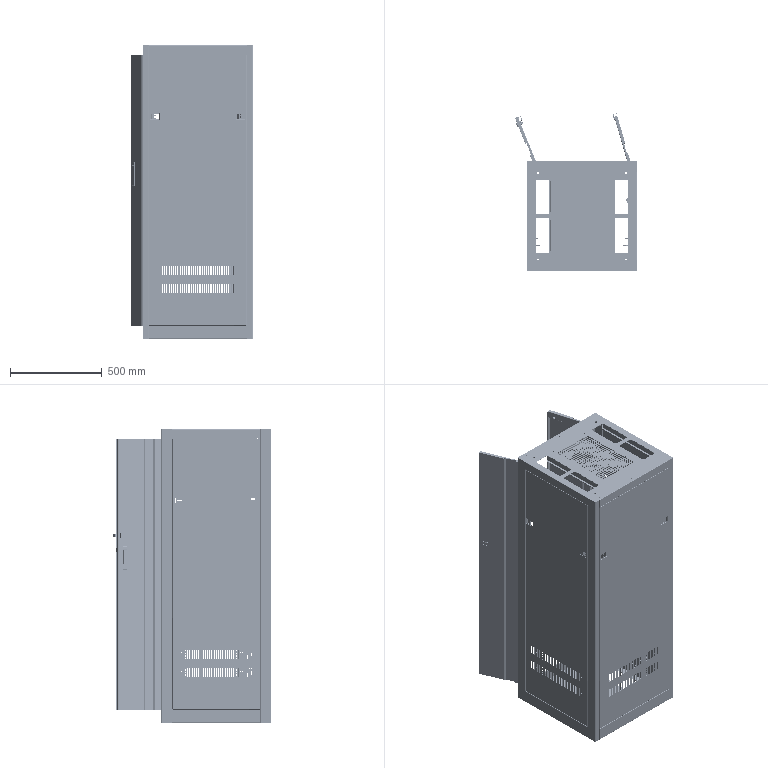Assembly | SolidWorks | mm | 61 component files | 61 solids | 10050 faces | box 662.77 x 864.74 x 1600 mm | volume 9328341 mm3 | plane 8344 | cylinder 1611 | spline 57 | sphere 16 | torus 14 | cone 8 | commonest cylinder face diameters 6 x533 2 x236 6.5 x162 1 x128 5 x74 9.2 x64 6.1 x52 4.5 x28
Bill of materials:
Base | 1 |  | Square, tray-like sheet-metal base plate. Formed channel walls run along two opposite edges and stop short of the corners, leaving gaps. The base has two long rounded-rectangle cutouts, round holes near the corners and small pierced holes.
Bracket1 | 4 |  | Long, straight Z-section profile of uniform cross-section: two parallel flanges joined by a web, with rounded bends.
Column | 4 |  | Long, slender formed sheet-metal profile with a multi-bend, stepped hat- or omega-like open cross-section. It has a row of small holes along its length and small notched tabs at one end.
FanMountingPlate | 1 |  | Rectangular, shallow open tray or box with vertical side walls and outward perimeter flanges. The base has two large circular cutouts, a small square cutout between them, and round holes.
2 | 1 |  | Long, narrow sheet-metal strip formed into a shallow channel (C/U) profile. The web has a repeating pattern of small square holes with adjacent slots along the full length.
CopperBarFixingClamp | 2 |  | Compact rectangular block with one rounded end. A deep slot along its length splits it into two parallel jaws (clevis- or fork-like), and a round through-hole passes across both jaws near the rounded end.
GroundingCopperBar | 1 |  | Very thin, flat rectangular plate or sheet panel, elongated in one direction, with tiny features along the long edges.
SC16-6 | 1 |  | Barrel-and-tongue lug-like part: a hollow cylindrical barrel joined through an offset transition to a flat rectangular tongue with rounded corners and one round through-hole.
GuidePlate | 4 |  | Long, straight formed rail with a stepped, hat-like cross-section and offset flanges. A row of square holes runs along the central raised section, and round holes sit near each end of both flanges.
Bolt | 2 |  | Solid round rod bent into a U or hairpin shape with two parallel legs of unequal length. The shorter leg has a circumferential groove or step near its end.
Bracket | 2 |  | Formed sheet-metal U or C bracket: a rectangular web with two parallel flanges bent at rounded corners. One flange has a round hole; each flange has a stepped notch giving a narrower tab at its free end.
EndCap1 | 2 |  | Long, formed sheet-metal channel with a multi-bend open profile (C-section with an extra offset return lip). The flanges have notched or stepped edges, there is a rectangular slot in the web near one end, and a small semicircular notch or hole sits at one end.
EndCap2 | 2 |  | Long, narrow formed sheet-metal channel or rail. It has an open, roughly C/Z-shaped cross-section with flanges that are offset from each other, stepped notches along the flange edges, and a small rectangular slot in the web near one end.
LeftDoor | 1 |  | Long thin-walled profile with a constant cross-section. The end view shows a multi-bend zigzag of mostly straight segments with short hooked returns at both ends. A small protruding rib or tab runs along one segment near one end.
LockWeldBracket | 1 |  | Hat-shaped (omega-profile) bent strip bracket. A central flat web has three round holes in a triangular pattern. Two side walls stand perpendicular to the web, and two outward-turned end flanges are coplanar with each other.
PadlockBracket | 1 |  | L-shaped bent plate bracket with two legs at roughly 90 degrees and a rounded bend. The shorter leg has three small round holes in a triangular pattern. The longer leg ends in a fully rounded end with one larger round hole.
Pin | 8 |  | Solid revolved pin or plug-like part. From one end it has a short cylindrical head, then a wider thin circular collar, then a cylindrical shank ending in a hemispherical (domed) tip.
Spring | 2 |  | Helical coil spring made of round wire. It has about 11 coils of uniform diameter, an open pitch, and plain cut ends that are not closed.
RearDoor | 1 |  | Thin flat rectangular panel. It has two small rectangular cutouts near the side edges toward one end, and two parallel rows of narrow elongated slots (vent-like) near the other end. Small round holes are visible on one narrow edge face.
ReinforcementPlate1 | 1 |  | Flat plate bracket whose outline has one chamfered (diagonally cut) corner. Two rectangular tabs on adjacent edges are bent up at about 90 degrees. The plate has two large round holes, several smaller round holes, and narrow rectangular slots cut in from the edges.
ReinforcementPlate2 | 1 |  | Flat plate bracket with one chamfered corner. Two rectangular tabs on adjacent edges are bent up at about 90 degrees. The plate has two large round holes, several smaller round holes, and narrow edge slots. The layout appears mirrored relative to unnamed part.
Latch | 1 |  | Bent flat strip with an S/Z-shaped jog made by two rounded bends, so the end segments are offset and run in parallel directions. One end segment has a square through-hole oriented as a diamond.
LockBody | 1 |  | Compact, blocky multi-feature part. A thin base plate or flange strip carries two raised rectangular blocks separated by a gap. One block has a chamfered or angled top. Shallow rectangular recesses are on the top face, and small round holes or bosses are on the side faces.
LowerRod | 1 |  | Long narrow flat strip with two jogged offsets along its length, so the middle and end sections step sideways. A small tab or barb-like protrusion sits at one end. The view along the length shows a T-shaped head over a narrower neck and a wider body.
UpperRod | 1 |  | Long, narrow flat strip with a joggle (offset bend) near one end. A short headed pin or stud sticks out from the face near the offset end.
LowerLinkRod1 | 1 |  | Very slender flat strip with a joggle near one end. One end has a small square hole and the other end is rounded with a small round hole.
Roller | 4 |  | Flat circular disc with one concentric through-hole, shaped like a washer or spacer. The outer edge appears slightly rounded or chamfered.
UpperLinkRod | 1 |  | Long, slender flat strip similar to a link or strap. It has a joggle near one end, a rounded end with a small round hole, and a small square hole at the opposite end.
RightDoor | 1 |  | Long formed sheet-metal profile. In cross-section it has a long inclined web with stepped jogs and short return flanges at both ends. The web has a rectangular slot and a small cylindrical pin.
SideDoor | 2 |  | Tall rectangular thin panel with narrow folded edges. It has two small rectangular cutouts near the top, two rows of parallel slotted vents near the bottom, and round holes on the narrow edge flanges near each end.
SmallColumn | 4 |  | Long, slender bent-strip profile with a stepped Z/hat-like cross-section and rounded bends. A regular row of small holes and slots runs along its full length.
TopBase | 1 |  | Square-ish shallow tray or cover plate with folded side flanges. The center has a field of square perforations arranged in a grid. Four large rounded-rectangular cutouts sit near the sides, along with corner round holes and many small holes.
Mates:
1. coincident | Base-1 face at (312.828, 200.023, 0) dir (0, 0, 1) | ReinforcementPlate1-1 face at (-259.672, -298.477, 0) dir (0, 0, -1)
2. coincident | Base-1 face at (312.828, 200.023, 0) dir (0, 0, 1) | ReinforcementPlate2-1 face at (214.328, -372.477, 0) dir (0, 0, -1)
3. coincident | Base-1 face at (-285.672, 141.523, 0) dir (-1, 0, 0) | Column-2 face at (-285.672, -398.477, -1.5) dir (-1, 0, 0)
4. coincident | Base-1 face at (312.828, 200.023, -1.5) dir (0, 0, -1) | Column-2 face at (-283.172, -339.977, -1.5) dir (0, 0, -1)
5. coincident | Base-1 face at (282.328, -398.477, 0) dir (0, -1, 0) | Column-2 face at (-285.672, -398.477, -1.5) dir (0, -1, 0)
6. coincident | Base-1 face at (282.328, -398.477, 0) dir (0, -1, 0) | Column-1 face at (314.328, -398.477, 1598.5) dir (0, -1, 0)
7. coincident | Base-1 face at (314.328, -338.477, 68.5) dir (1, 0, 0) | Column-1 face at (314.328, -398.477, 1598.5) dir (1, 0, 0)
8. coincident | Base-1 face at (312.828, 200.023, -1.5) dir (0, 0, -1) | Column-1 face at (283.828, -395.977, -1.5) dir (0, 0, -1)
9. coincident | Base-1 face at (314.328, -338.477, 68.5) dir (1, 0, 0) | Column-4 face at (314.328, 201.523, -1.5) dir (1, 0, 0)
10. coincident | Base-1 face at (312.828, 200.023, -1.5) dir (0, 0, -1) | Column-4 face at (311.828, 143.023, -1.5) dir (0, 0, -1)
11. coincident | Base-1 face at (282.328, 201.523, 0) dir (0, 1, 0) | Column-4 face at (314.328, 201.523, -1.5) dir (0, 1, 0)
12. coincident | Base-1 face at (282.328, 201.523, 0) dir (0, 1, 0) | Column-3 face at (-285.672, 201.523, 1598.5) dir (0, 1, 0)
13. coincident | Base-1 face at (-285.672, 141.523, 0) dir (-1, 0, 0) | Column-3 face at (-285.672, 201.523, 1598.5) dir (-1, 0, 0)
14. coincident | Base-1 face at (312.828, 200.023, -1.5) dir (0, 0, -1) | Column-3 face at (-283.172, 200.023, -1.5) dir (0, 0, -1)
15. coincident | Column-2 face at (-253.672, -372.477, -1.5) dir (0, 1, 0) | ReinforcementPlate1-1 face at (-235.672, -372.477, 3) dir (0, -1, 0)
16. coincident | Column-2 face at (-259.672, -338.477, -1.5) dir (1, 0, 0) | ReinforcementPlate1-1 face at (-259.672, -322.477, 3) dir (-1, 0, 0)
17. coincident | Column-1 face at (288.328, -338.477, 1598.5) dir (-1, 0, 0) | ReinforcementPlate2-1 face at (288.328, -322.477, 3) dir (1, 0, 0)
18. coincident | Column-1 face at (282.328, -372.477, 1598.5) dir (0, 1, 0) | ReinforcementPlate2-1 face at (288.328, -372.477, 3) dir (0, -1, 0)
19. coincident | Column-2 face at (-255.172, -395.977, 1598.5) dir (0, 0, 1) | TopBase-1 face at (-284.172, 200.023, 1598.5) dir (0, 0, 1)
20. coincident | Column-2 face at (-285.672, -398.477, -1.5) dir (0, -1, 0) | TopBase-1 face at (282.328, -398.477, 1597) dir (0, -1, 0)
21. coincident | Column-2 face at (-285.672, -398.477, -1.5) dir (-1, 0, 0) | TopBase-1 face at (-285.672, -338.477, 1548.5) dir (-1, 0, 0)
22. coincident | Column-3 face at (-259.672, 141.523, 1598.5) dir (1, 0, 0) | GuidePlate-5 face at (-259.672, 152.023, 1383.5) dir (-1, 0, 0)
23. distance | GuidePlate-5 face at (-259.672, -347.977, 1414.5) dir (0, -1, 0) | Column-2 face at (-285.672, -339.977, -1.5) dir (0, -1, 0)
24. distance | GuidePlate-5 plane at (-239.672, -97.977, 1398.5) dir (0, 0, -1) | TopBase-1 face at (-284.172, 200.023, 1598.5) dir (0, 0, 1)
25. coincident | Column-1 face at (288.328, -338.477, 1598.5) dir (-1, 0, 0) | GuidePlate-3 face at (288.328, -347.977, 1413.5) dir (1, 0, 0)
26. coincident | GuidePlate-5 face at (-242.172, -347.977, 1412) dir (0, -1, 0) | GuidePlate-3 face at (270.828, -347.977, 1385) dir (0, -1, 0)
27. distance | GuidePlate-3 plane at (268.328, -97.977, 1398.5) dir (0, 0, -1) | TopBase-1 face at (-284.172, 200.023, 1598.5) dir (0, 0, 1)
28. coincident | GuidePlate-3 face at (268.328, -347.977, 1413.5) dir (-1, 0, 0) | SmallColumn-1 face at (268.328, 121.523, 39.165) dir (1, 0, 0)
29. distance | SmallColumn-1 face at (268.328, 121.523, 39.165) dir (0, 1, 0) | Column-4 face at (314.328, 201.523, -1.5) dir (0, 1, 0)
30. coincident | GuidePlate-6 face at (-239.672, 152.023, 513.5) dir (1, 0, 0) | SmallColumn-2 face at (-239.672, 121.523, 1499.165) dir (-1, 0, 0)
31. coincident | SmallColumn-1 face at (268.328, 121.523, 39.165) dir (0, 1, 0) | SmallColumn-2 face at (-239.672, 121.523, 1499.165) dir (0, 1, 0)
32. coincident | SmallColumn-1 face at (265.328, 83.523, 39.165) dir (0, 0, -1) | SmallColumn-2 face at (-236.672, 119.523, 39.165) dir (0, 0, -1)
33. coincident | TopBase-1 face at (-284.172, 200.023, 1597) dir (0, 0, -1) | FanMountingPlate-1 face at (145.818, -295.977, 1597) dir (0, 0, 1)
34. coincident | GuidePlate-4 face at (268.328, -347.977, 513.5) dir (-1, 0, 0) | SmallColumn-5 face at (268.328, -258.477, 1499.165) dir (1, 0, 0)
35. coincident | SmallColumn-1 face at (253.328, 80.523, 39.165) dir (0, 0, -1) | SmallColumn-5 face at (253.328, -220.477, 39.165) dir (0, 0, -1)
36. distance | SmallColumn-1 face at (250.328, 61.523, 39.165) dir (0, -1, 0) | SmallColumn-5 face at (268.328, -258.477, 1499.165) dir (0, -1, 0)
37. coincident | GuidePlate-6 face at (-239.672, 152.023, 513.5) dir (1, 0, 0) | SmallColumn-6 face at (-239.672, -258.477, 39.165) dir (-1, 0, 0)
38. coincident | SmallColumn-5 face at (268.328, -258.477, 1499.165) dir (0, -1, 0) | SmallColumn-6 face at (-239.672, -258.477, 39.165) dir (0, -1, 0)
39. coincident | SmallColumn-5 face at (265.328, -256.477, 39.165) dir (0, 0, -1) | SmallColumn-6 face at (-236.672, -220.477, 39.165) dir (0, 0, -1)
40. coincident | FixedStrip-4 face at (268.328, -338.477, 1535.585) dir (1, 0, 0) | GuidePlate-4 face at (268.328, -347.977, 513.5) dir (-1, 0, 0)
41. concentric | TopBase-1 face at (134.328, 106.523, 1607) dir (0, 0, -1) r 3.05 | FanMountingPlate-1 face at (134.328, 106.523, 1587) dir (0, 0, 1) r 2.25
42. concentric | TopBase-1 face at (-105.672, 106.523, 1607) dir (0, 0, -1) r 3.05 | FanMountingPlate-1 face at (-105.672, 106.523, 1587) dir (0, 0, 1) r 2.25
43. coincident | TopBase-1 face at (-284.172, 200.023, 1597) dir (0, 0, -1) | Bracket1-1 face at (275.828, -298.477, 1597) dir (0, 0, 1)
44. coincident | TopBase-1 face at (274.328, -120.977, 1598.5) dir (-1, 0, 0) | Bracket1-1 face at (274.328, -298.477, 1566) dir (-1, 0, 0)
45. coincident | TopBase-1 face at (264.328, -298.477, 1598.5) dir (0, 1, 0) | Bracket1-1 face at (276.828, -298.477, 1597) dir (0, -1, 0)
46. coincident | TopBase-1 face at (-284.172, 200.023, 1597) dir (0, 0, -1) | Bracket1-5 face at (184.328, 101.523, 1597) dir (0, 0, 1)
47. coincident | TopBase-1 face at (184.328, 91.523, 1598.5) dir (1, 0, 0) | Bracket1-5 face at (184.328, 101.523, 1597) dir (1, 0, 0)
48. coincident | Bracket1-1 face at (276.828, -298.477, 1597) dir (0, -1, 0) | Bracket1-5 face at (181.828, -298.477, 1595.5) dir (0, -1, 0)
49. coincident | Base-1 face at (-284.172, -338.477, 68.5) dir (0, 0, 1) | SideDoorAssembly-1/Pin-1 face at (-275.172, -288.477, 68.5) dir (0, 0, -1)
50. concentric | Base-1 face at (-275.172, -288.477, -1.501) dir (0, 0, 1) r 3.25 | SideDoorAssembly-1/Pin-1 face at (-275.172, -288.477, 72.2) dir (0, 0, 1) r 3
51. concentric | Base-1 face at (-275.172, 91.523, -1.501) dir (0, 0, 1) r 3.25 | SideDoorAssembly-1/Pin-2 face at (-275.172, 91.523, 72.2) dir (0, 0, 1) r 3
52. coincident | Base-1 face at (282.328, -396.977, 68.5) dir (0, 0, 1) | RearDoorAssembly-1/Pin-2 face at (-175.672, -387.977, 68.5) dir (0, 0, -1)
53. concentric | RearDoorAssembly-1/Pin-2 face at (-175.672, -387.977, 72.2) dir (0, 0, 1) r 3 | Base-1 face at (-175.672, -387.977, -1.501) dir (0, 0, 1) r 3.25
54. concentric | RearDoorAssembly-1/Pin-1 face at (204.328, -387.977, 72.2) dir (0, 0, 1) r 3 | Base-1 face at (204.328, -387.977, -1.501) dir (0, 0, 1) r 3.25
55. coincident | Base-1 face at (-253.672, 200.023, 68.5) dir (0, 0, 1) | LeftDoorAssembly-1/Pin-1 face at (275.828, 196.273, 68.5) dir (0, 0, -1)
56. concentric | Base-1 face at (275.828, 196.273, -1.501) dir (0, 0, 1) r 3.25 | LeftDoorAssembly-1/Pin-1 face at (275.828, 196.273, 72.2) dir (0, 0, 1) r 3
57. coincident | Base-1 face at (-253.672, 200.023, 68.5) dir (0, 0, 1) | RightDoorAssembly-1/Pin-1 face at (-247.172, 196.273, 68.5) dir (0, 0, -1)
58. concentric | Base-1 face at (-247.172, 196.273, -1.501) dir (0, 0, 1) r 3.25 | RightDoorAssembly-1/Pin-1 face at (-247.172, 196.273, 72.2) dir (0, 0, 1) r 3
59. coincident | GuidePlate-4 face at (268.328, -347.977, 513.5) dir (-1, 0, 0) | GroundingSystem-1/CopperBarFixingClamp-2 face at (268.328, -2.944, 207.092) dir (1, 0, 0)
60. parallel | Column-4 face at (314.328, 201.523, -1.5) dir (0, 1, 0) | GroundingSystem-1/GroundingCopperBar-1 face at (266.828, -4.444, 1517.775) dir (0, 1, 0)
61. parallel | Column-1 face at (314.328, -398.477, 1598.5) dir (0, -1, 0) | FixedStrip-4 face at (268.328, -258.477, 1535.585) dir (0, 1, 0)
62. coincident | Base-1 face at (312.828, 141.523, 68.5) dir (0, 0, 1) | SideDoorAssembly-2/Pin-2 face at (303.828, -288.477, 68.5) dir (0, 0, -1)
63. concentric | Base-1 face at (303.828, -288.477, -1.501) dir (0, 0, 1) r 3.25 | SideDoorAssembly-2/Pin-2 face at (303.828, -288.477, 72.2) dir (0, 0, 1) r 3
64. concentric | Base-1 face at (303.828, 91.523, -1.501) dir (0, 0, 1) r 3.25 | SideDoorAssembly-2/Pin-1 face at (303.828, 91.523, 72.2) dir (0, 0, 1) r 3
65. coincident | GroundingCopperBar-1 face at (677.112, 63.748, 2) dir (0, 0, 1) | SC16-6-1 face at (-691.244, 51.356, 2) dir (0, 0, -1)
66. concentric | GroundingCopperBar-1 face at (-697.888, 57.748, 2) dir (0, 0, 1) r 2.1 | SC16-6-1 face at (-697.888, 57.748, -8.6) dir (0, 0, 1) r 3.25
67. coincident | GroundingCopperBar-1 face at (677.112, 63.748, 2) dir (0, 0, 1) | CopperBarFixingClamp-1 face at (-660.994, 51.748, 2) dir (0, 0, -1)
68. coincident | GroundingCopperBar-1 face at (-722.888, 51.748, -2) dir (0, -1, 0) | CopperBarFixingClamp-1 face at (-660.994, 51.748, 2) dir (0, 1, 0)
69. coincident | LeftDoor-1 face at (-466.038, 124.066, 900.924) dir (1, 0, 0) | EndCap2-1 face at (-466.038, -7.184, 899.724) dir (-1, 0, 0)
70. coincident | LeftDoor-1 face at (-465.745, 106.145, 900.924) dir (0, 0, 1) | EndCap2-1 face at (-451.038, -7.184, 900.924) dir (0, 0, 1)
71. coincident | LeftDoor-1 face at (-467.538, -7.184, 900.924) dir (0, 1, 0) | EndCap2-1 face at (-453.238, -7.184, 898.724) dir (0, -1, 0)
72. coincident | LeftDoor-1 face at (-466.038, 124.066, 900.924) dir (1, 0, 0) | EndCap1-1 face at (-466.038, -7.184, -576.076) dir (-1, 0, 0)
73. coincident | LeftDoor-1 face at (-465.038, 255.316, -576.076) dir (0, 0, -1) | EndCap1-1 face at (-451.038, -7.184, -576.076) dir (0, 0, -1)
74. coincident | LeftDoor-1 face at (-467.538, -7.184, 900.924) dir (0, 1, 0) | EndCap1-1 face at (-452.238, -7.184, -573.876) dir (0, -1, 0)
75. coincident | EndCap2-1 face at (-451.038, -7.184, 900.924) dir (0, 0, 1) | Pin-1 face at (-462.788, -3.934, 900.924) dir (0, 0, -1)
76. concentric | EndCap2-1 face at (-462.788, -3.934, 900.924) dir (0, 0, -1) r 3.25 | Pin-1 face at (-462.788, -3.934, 898.924) dir (0, 0, -1) r 4
77. coincident | LeftDoor-1 face at (-466.038, 124.066, 900.924) dir (1, 0, 0) | Bracket-1 face at (-466.038, -7.184, -563.876) dir (-1, 0, 0)
78. coincident | LeftDoor-1 face at (-467.538, -7.184, 900.924) dir (0, 1, 0) | Bracket-1 face at (-463.838, -7.184, -527.276) dir (0, -1, 0)
79. distance | EndCap1-1 face at (-451.038, -7.184, -576.076) dir (0, 0, -1) | Bracket-1 face at (-464.838, -7.184, -565.076) dir (0, 0, -1)
80. concentric | Bracket-1 face at (-456.538, 19.956, -525.076) dir (0, 0, -1) r 3.25 | Bolt-1 face at (-456.538, 19.956, -518.678) dir (0, 0, -1) r 3
81. tangent | Bolt-1 face at (-456.538, 19.956, -518.678) dir (0, 0, -1) r 3 | Spring-1 face at (-452.759, 20.301, -528.804) dir (1, 0, 0)
82. coincident | LeftDoor-1 face at (-466.038, 124.066, 900.924) dir (1, 0, 0) | LockWeldBracket-1 face at (-466.038, 255.316, -34.076) dir (-1, 0, 0)
83. coincident | LockWeldBracket-1 face at (-447.038, 255.316, -64.076) dir (1, 0, 0) | PadlockBracket-1 face at (-447.038, 271.316, -59.076) dir (-1, 0, 0)
84. concentric | PadlockBracket-1 face at (-455.038, 243.316, -43.076) dir (1, 0, 0) r 2.25 | LockWeldBracket-1 face at (-457.038, 243.316, -43.076) dir (1, 0, 0) r 2.25
85. concentric | LockWeldBracket-1 face at (-457.038, 243.316, -55.076) dir (1, 0, 0) r 2.25 | PadlockBracket-1 face at (-455.038, 243.316, -55.076) dir (1, 0, 0) r 2.25
86. coincident | LeftDoor-1 face at (-467.538, 255.316, 900.924) dir (0, -1, 0) | LockWeldBracket-1 face at (-449.048, 255.316, -62.076) dir (0, 1, 0)
87. distance | LockWeldBracket-1 plane at (-464.038, 247.316, -49.076) dir (0, 0, 1) | EndCap2-1 face at (-451.038, -7.184, 900.924) dir (0, 0, 1)
88. concentric | EndCap1-1 face at (-462.788, -3.934, -536.076) dir (0, 0, -1) r 3.25 | Bolt-1 face at (-462.788, -3.934, -518.678) dir (0, 0, -1) r 3
89. coincident | RearDoor-1 face at (-779.54, -7595.793, 17.5) dir (-1, 0, 0) | Pin-1 face at (-779.54, 246.207, 8.8) dir (1, 0, 0)
90. concentric | RearDoor-1 face at (697.46, 246.207, 8.8) dir (-1, 0, 0) r 3.25 | Pin-1 face at (-777.54, 246.207, 8.8) dir (1, 0, 0) r 3.25
91. coincident | RightDoor-1 face at (-125.665, -23.878, 816.813) dir (1, 0, 0) | EndCap1-1 face at (-125.665, -155.128, -660.187) dir (-1, 0, 0)
92. coincident | RightDoor-1 face at (-127.165, -155.128, 816.813) dir (0, 1, 0) | EndCap1-1 face at (-112.865, -155.128, -621.387) dir (0, -1, 0)
93. coincident | RightDoor-1 face at (-124.665, 107.372, -660.187) dir (0, 0, -1) | EndCap1-1 face at (-110.665, -155.128, -660.187) dir (0, 0, -1)
94. coincident | RightDoor-1 face at (-125.665, -23.878, 816.813) dir (1, 0, 0) | EndCap2-1 face at (-125.665, -155.128, 815.613) dir (-1, 0, 0)
95. coincident | RightDoor-1 face at (-125.372, -41.8, 816.813) dir (0, 0, 1) | EndCap2-1 face at (-110.665, -155.128, 816.813) dir (0, 0, 1)
96. coincident | RightDoor-1 face at (-127.165, -155.128, 816.813) dir (0, 1, 0) | EndCap2-1 face at (-112.865, -155.128, 814.613) dir (0, -1, 0)
97. coincident | EndCap1-1 face at (-110.665, -155.128, -660.187) dir (0, 0, -1) | Pin-1 face at (-122.415, -151.878, -660.187) dir (0, 0, 1)
98. concentric | EndCap2-1 face at (-122.415, -151.878, 816.813) dir (0, 0, -1) r 3.25 | Pin-1 face at (-122.415, -151.878, -658.187) dir (0, 0, 1) r 3.25
99. coincident | RightDoor-1 face at (-125.665, -23.878, 816.813) dir (1, 0, 0) | Bracket-1 face at (-125.665, -155.128, 767.013) dir (-1, 0, 0)
100. coincident | RightDoor-1 face at (-127.165, -155.128, 816.813) dir (0, 1, 0) | Bracket-1 face at (-125.665, -155.128, 768.013) dir (0, -1, 0)
101. distance | Bracket-1 face at (-124.465, -155.128, 805.813) dir (0, 0, 1) | EndCap2-1 face at (-110.665, -155.128, 816.813) dir (0, 0, 1)
102. concentric | Bracket-1 face at (-116.165, -127.988, 765.813) dir (0, 0, -1) r 3.25 | Bolt-1 face at (-116.165, -127.988, 757.308) dir (0, 0, 1) r 3
103. coincident | RightDoor-1 face at (-127.165, -23.878, 816.813) dir (-1, 0, 0) | LinkRodLock-1/Lock-1/LockBody-1 face at (-127.165, 52.872, 101.313) dir (1, 0, 0)
104. coincident | RightDoor-1 face at (-117.165, 81.372, 105.313) dir (0, -1, 0) | LinkRodLock-1/Lock-1/LockBody-1 face at (-111.165, 81.372, 228.313) dir (0, 1, 0)
105. coincident | RightDoor-1 face at (-117.165, 81.372, 230.313) dir (0, 0, -1) | LinkRodLock-1/Lock-1/LockBody-1 face at (-127.165, 52.872, 230.313) dir (0, 0, 1)
106. concentric | EndCap2-1 face at (-122.415, -151.878, 816.813) dir (0, 0, -1) r 3.25 | Bolt-1 face at (-122.415, -151.878, 757.308) dir (0, 0, 1) r 3
107. coincident | Bolt-1 axis at (-116.165, -127.988, 813.158) dir (0, 0, 1) | Spring-1 plane at (-116.165, -127.988, 769.446) dir (-0.9148, 0.4039, 0)
108. coincident | Bolt-1 axis at (-116.165, -127.988, 813.158) dir (0, 0, 1) | Spring-1 plane at (-116.165, -127.988, 769.446) dir (0.4039, 0.9148, 0)
109. coincident | UpperLinkRod-1 face at (-29.505, 554.743, 8.115) dir (1, 0, 0) | Lock-1/UpperRod-1 face at (-29.505, 122.87, -8.385) dir (-1, 0, 0)
110. tangent | UpperLinkRod-1 face at (-32.505, 142.377, 0.365) dir (0, -1, 0) | Lock-1/UpperRod-1 face at (-33.505, 139.627, -3.385) dir (1, 0, 0) r 2.75
111. tangent | Lock-1/UpperRod-1 face at (-33.505, 139.627, -3.385) dir (1, 0, 0) r 2.75 | UpperLinkRod-1 face at (-32.505, 142.377, -6.135) dir (0, 0, 1)
112. coincident | Lock-1/LowerRod-1 face at (-30.505, -76.615, -8.385) dir (1, 0, 0) | LowerLinkRod1-1 face at (-30.505, -717.488, 8.115) dir (-1, 0, 0)
113. tangent | Lock-1/LowerRod-1 face at (-26.505, -100.373, -3.385) dir (-1, 0, 0) r 2.75 | LowerLinkRod1-1 face at (-27.505, -97.623, -6.135) dir (0, -1, 0)
114. tangent | Lock-1/LowerRod-1 face at (-26.505, -100.373, -3.385) dir (-1, 0, 0) r 2.75 | LowerLinkRod1-1 face at (-27.505, -104.123, -6.135) dir (0, 0, 1)
115. parallel | Lock-1/LowerRod-1 face at (-32.262, -72.373, -8.385) dir (0, 0, -1) | LowerLinkRod1-1 face at (-27.505, -90.873, -8.885) dir (0, 0, -1)
116. parallel | Lock-1/UpperRod-1 face at (-27.748, 118.627, -8.385) dir (0, 0, -1) | UpperLinkRod-1 face at (-32.505, 129.127, -8.885) dir (0, 0, -1)
117. coincident | UpperLinkRod-1 face at (-29.505, 554.743, 8.115) dir (1, 0, 0) | Roller-1 face at (-29.505, 634.127, 9.115) dir (-1, 0, 0)
118. concentric | UpperLinkRod-1 face at (-32.505, 634.127, 9.115) dir (1, 0, 0) r 2.1 | Roller-1 face at (-25.505, 634.127, 9.115) dir (-1, 0, 0) r 2.05
119. coincident | UpperLinkRod-1 face at (-32.505, 554.743, 8.115) dir (-1, 0, 0) | Roller-2 face at (-32.505, 634.127, 9.115) dir (1, 0, 0)
120. concentric | UpperLinkRod-1 face at (-32.505, 634.127, 9.115) dir (1, 0, 0) r 2.1 | Roller-2 face at (-36.505, 634.127, 9.115) dir (1, 0, 0) r 2.05
121. coincident | LowerLinkRod1-1 face at (-30.505, -717.488, 8.115) dir (-1, 0, 0) | Roller-3 face at (-30.505, -796.873, 9.115) dir (1, 0, 0)
122. concentric | LowerLinkRod1-1 face at (-27.505, -796.873, 9.115) dir (-1, 0, 0) r 2.1 | Roller-3 face at (-34.505, -796.873, 9.115) dir (1, 0, 0) r 2.05
123. coincident | LowerLinkRod1-1 face at (-27.505, -717.488, 8.115) dir (1, 0, 0) | Roller-4 face at (-27.505, -796.873, 9.115) dir (-1, 0, 0)
124. concentric | LowerLinkRod1-1 face at (-27.505, -796.873, 9.115) dir (-1, 0, 0) r 2.1 | Roller-4 face at (-23.505, -796.873, 9.115) dir (-1, 0, 0) r 2.05
125. coincident | LockBody-1 face at (-26.291, 24.793, 17.5) dir (0, 0, 1) | Latch-1 face at (-19.791, 56.293, 17.5) dir (0, 0, -1)
126. coincident | LockBody-1 face at (-13.791, 51.95, 21.5) dir (0.7071, 0.7071, 0) | Latch-1 face at (-8.134, 46.293, 10.5) dir (-0.7071, -0.7071, 0)
127. coincident | LockBody-1 face at (-13.791, 51.95, 21.5) dir (-0.7071, 0.7071, 0) | Latch-1 face at (-19.448, 46.293, 10.5) dir (0.7071, -0.7071, 0)
128. coincident | LockBody-1 face at (-2.041, -19.109, 4.5) dir (-1, 0, 0) | UpperRod-1 face at (-2.041, 108.808, 5) dir (1, 0, 0)
129. distance | LockBody-1 face at (-2.041, -19.109, 4.5) dir (0, 0, 1) | UpperRod-1 face at (-6.041, 119.536, 5) dir (0, 0, -1)
130. coincident | LockBody-1 face at (-22.541, -19.109, 4.5) dir (-1, 0, 0) | LowerRod-1 face at (-22.541, 78.793, 5) dir (1, 0, 0)
131. distance | LockBody-1 face at (-25.541, -19.109, 15.5) dir (0, 0, -1) | LowerRod-1 face at (-24.337, 14.753, 15) dir (0, 0, 1)
132. distance | UpperRod-1 face at (-9.041, 141.293, 5) dir (0, 1, 0) | LockBody-1 axis at (-13.791, 46.293, 16.5) dir (0, 0, 1)
133. distance | LockBody-1 axis at (-13.791, 46.293, 16.5) dir (0, 0, 1) | LowerRod-1 face at (-16.041, -108.707, 5) dir (0, -1, 0)
134. coincident | SideDoor-1 face at (-670.694, -7573.146, 8.7) dir (-1, 0, 0) | Pin-1 face at (-670.694, 240.854, 0) dir (1, 0, 0)
135. concentric | SideDoor-1 face at (806.306, 240.854, 0) dir (-1, 0, 0) r 3.25 | Pin-1 face at (-668.694, 240.854, 0) dir (1, 0, 0) r 3